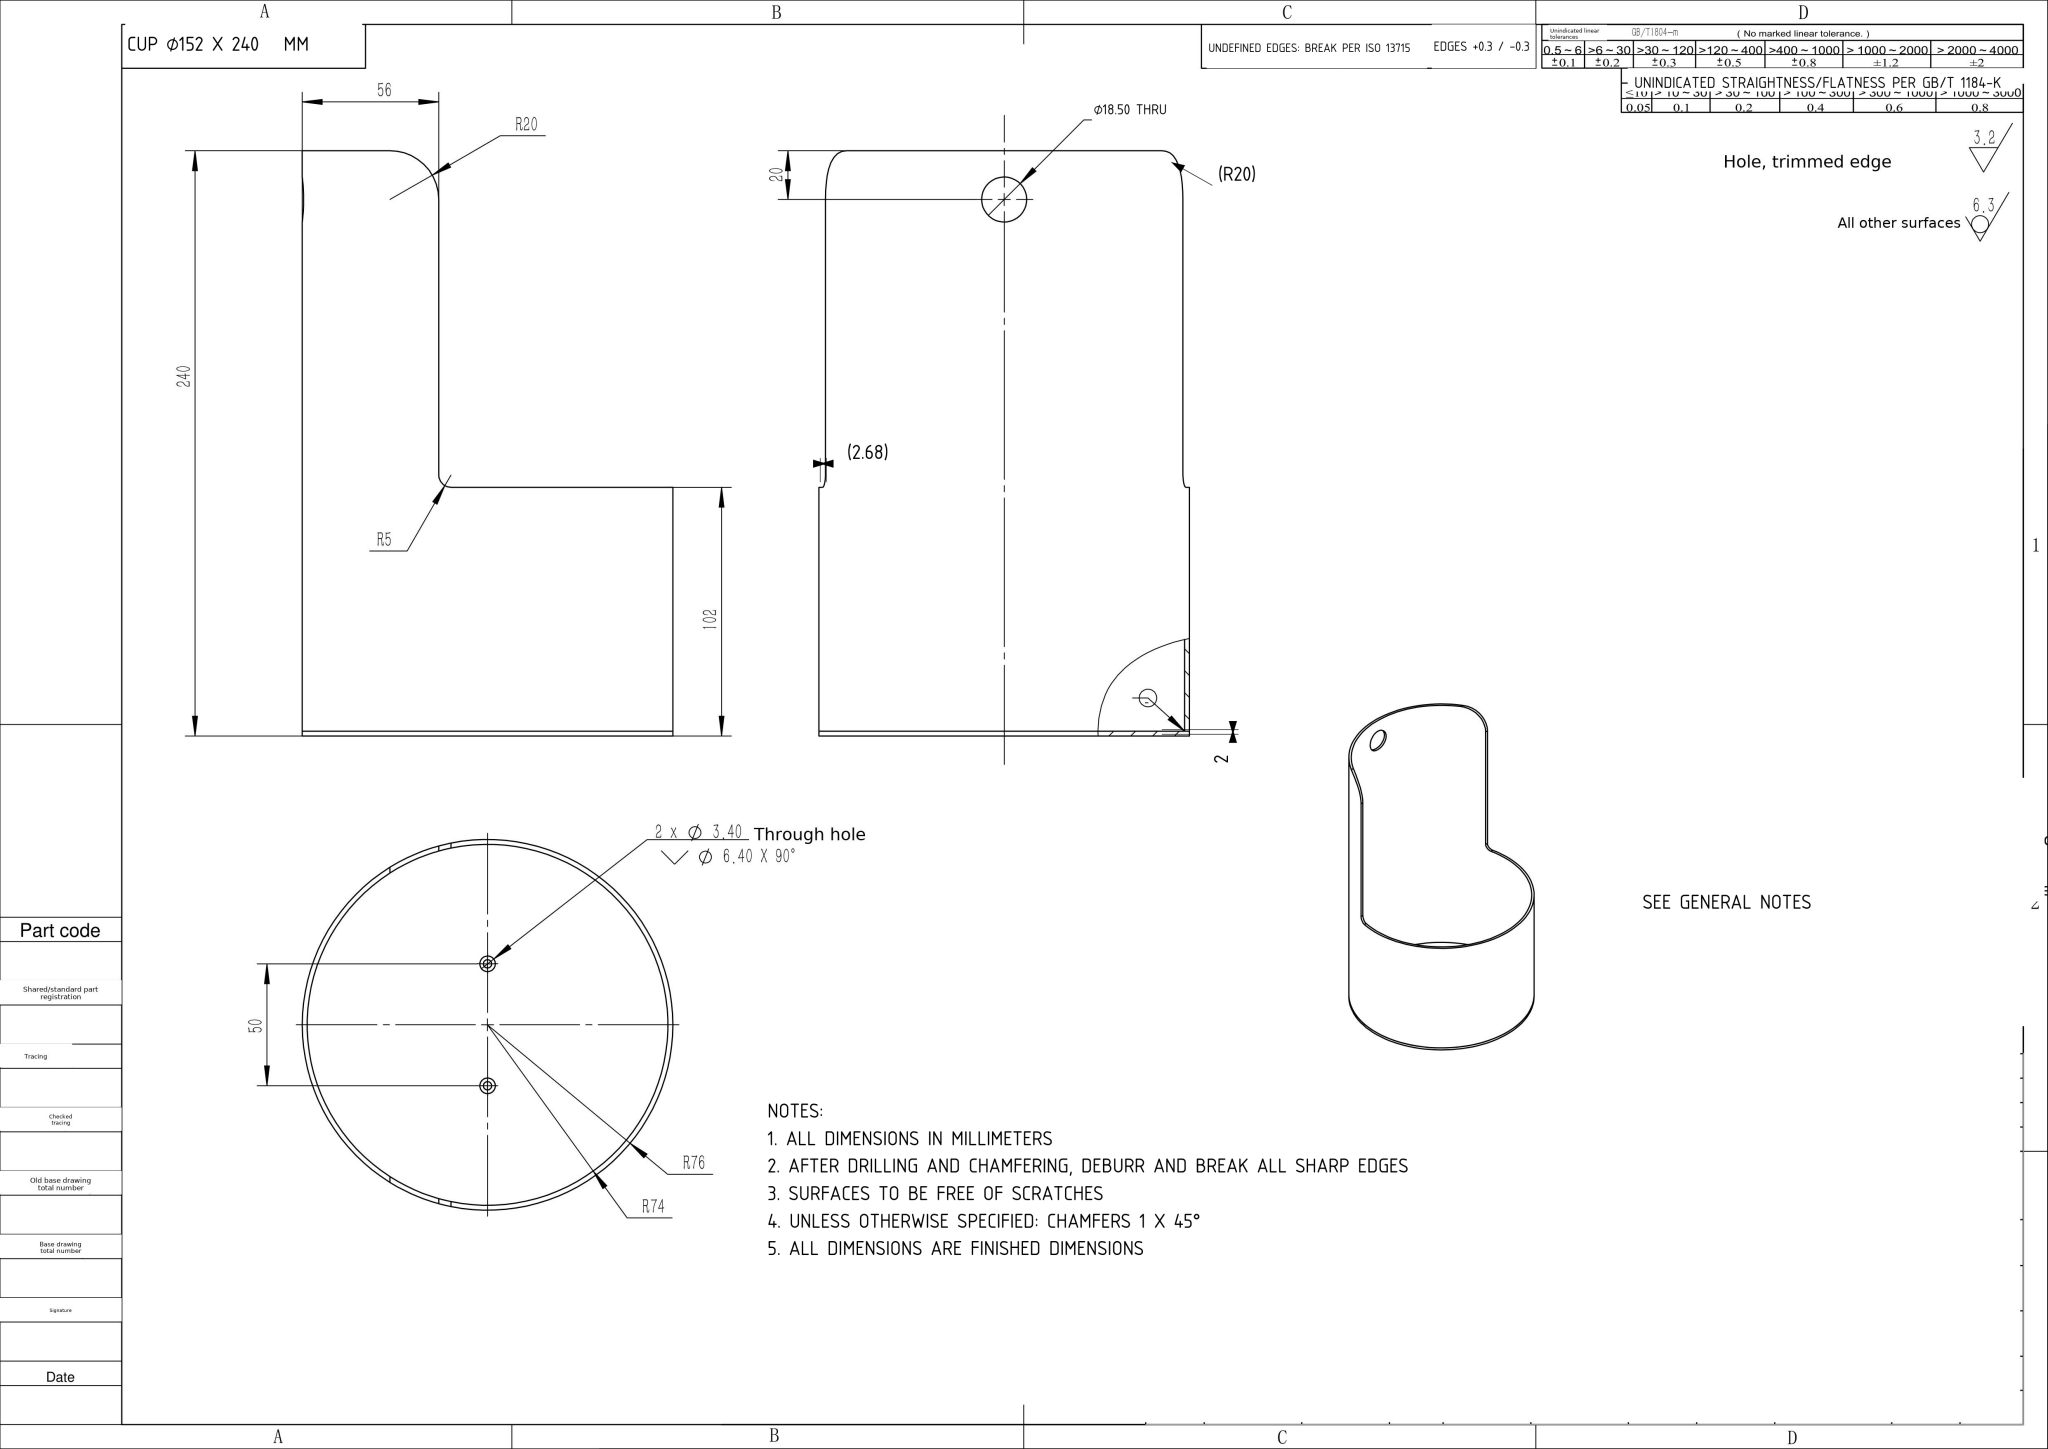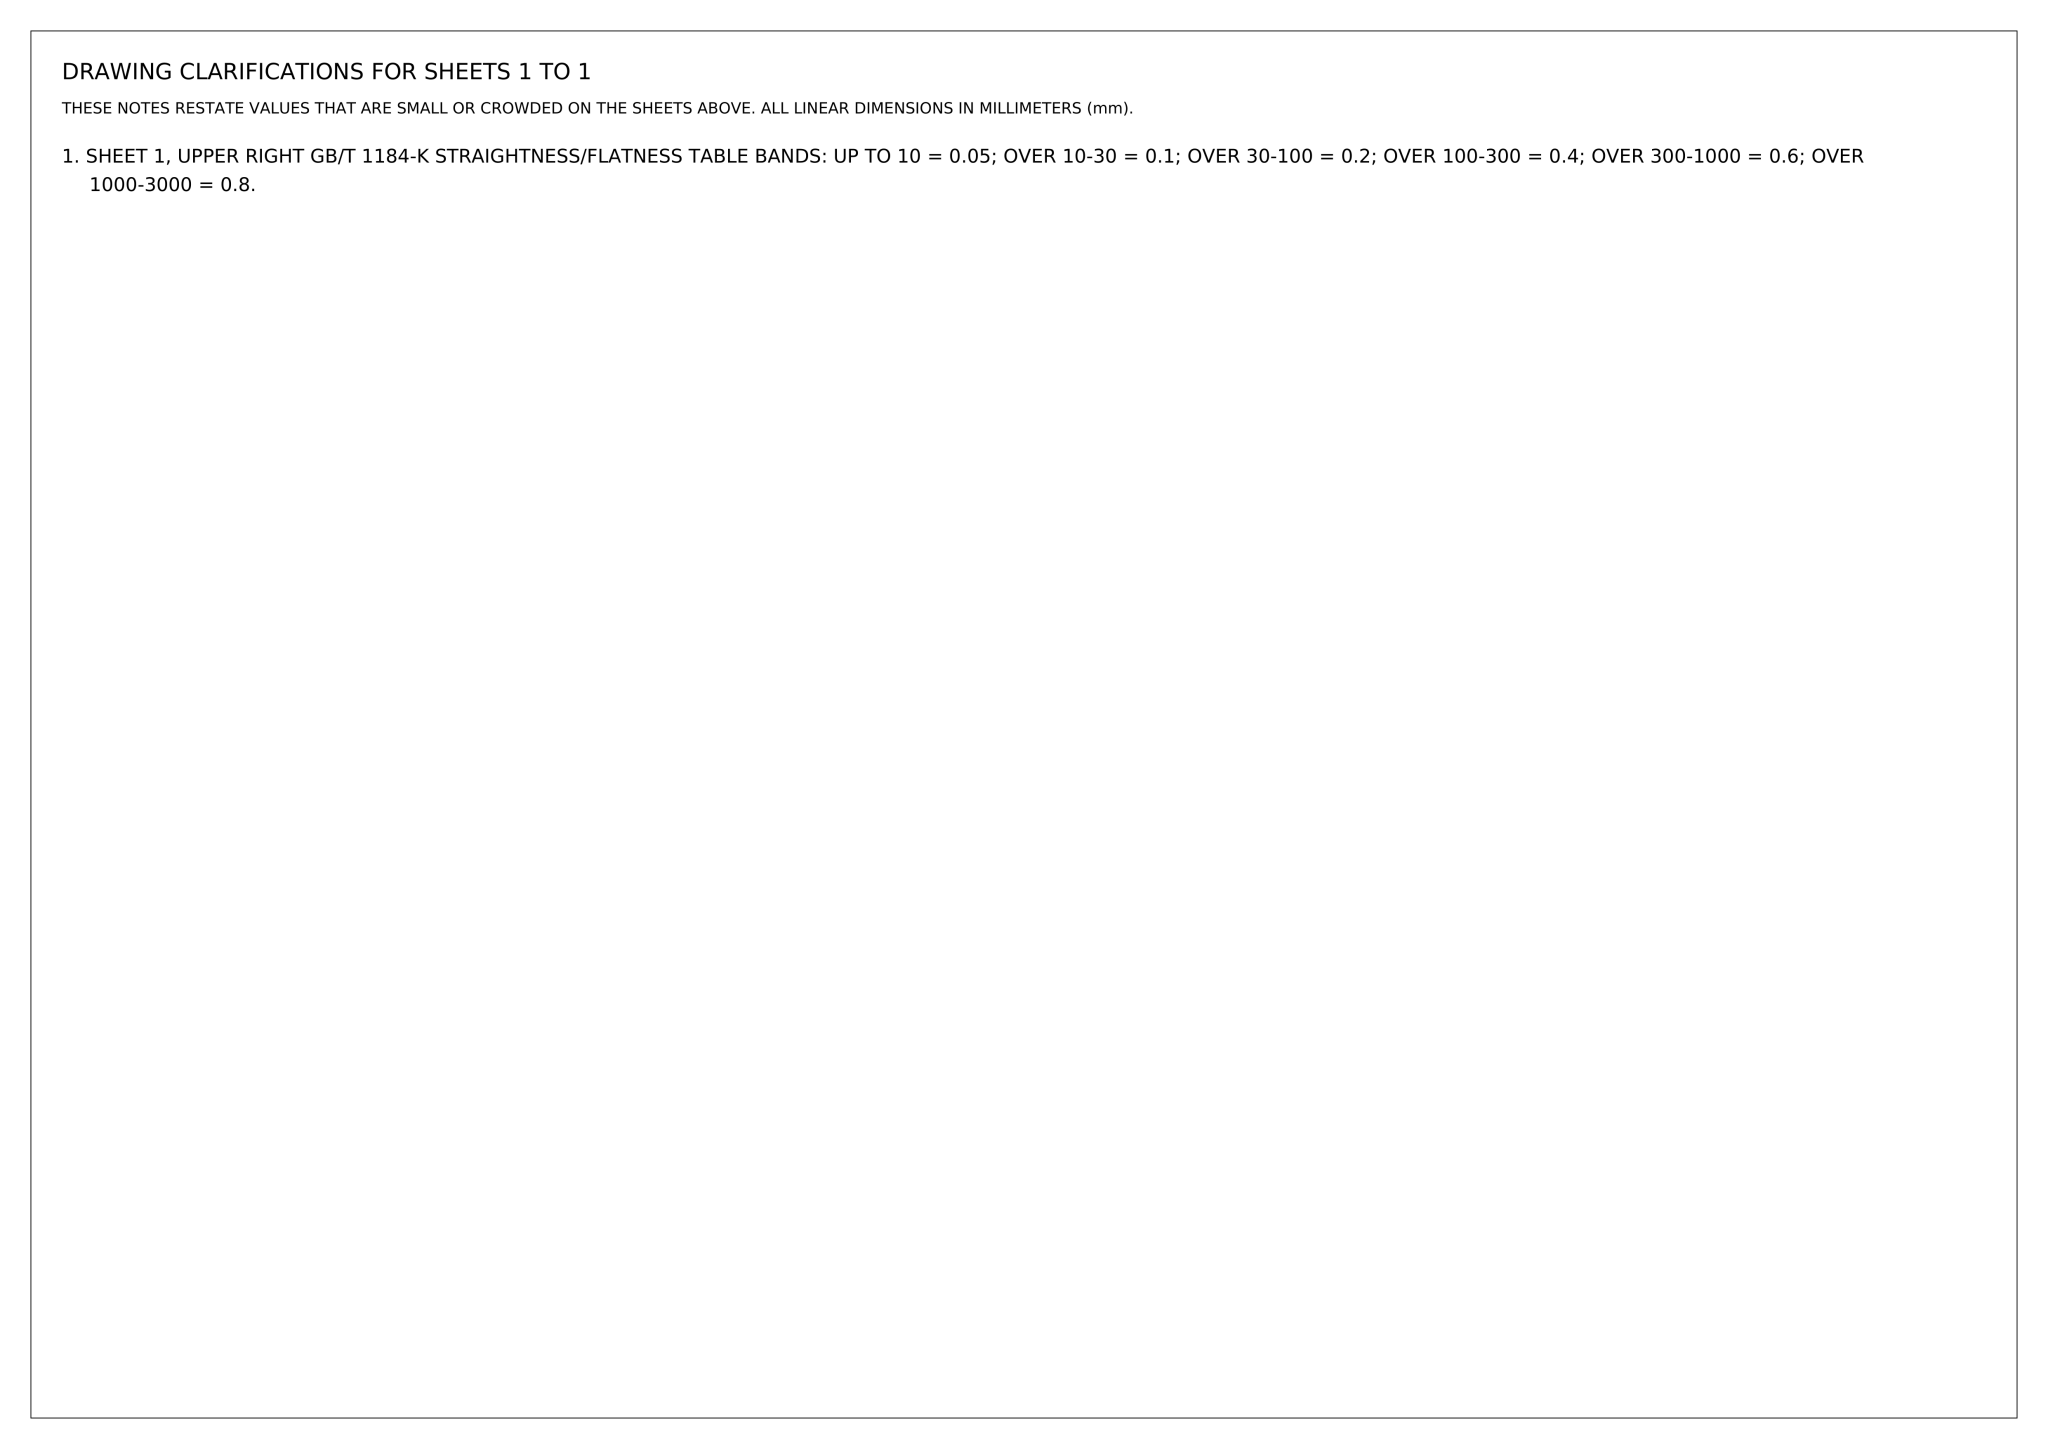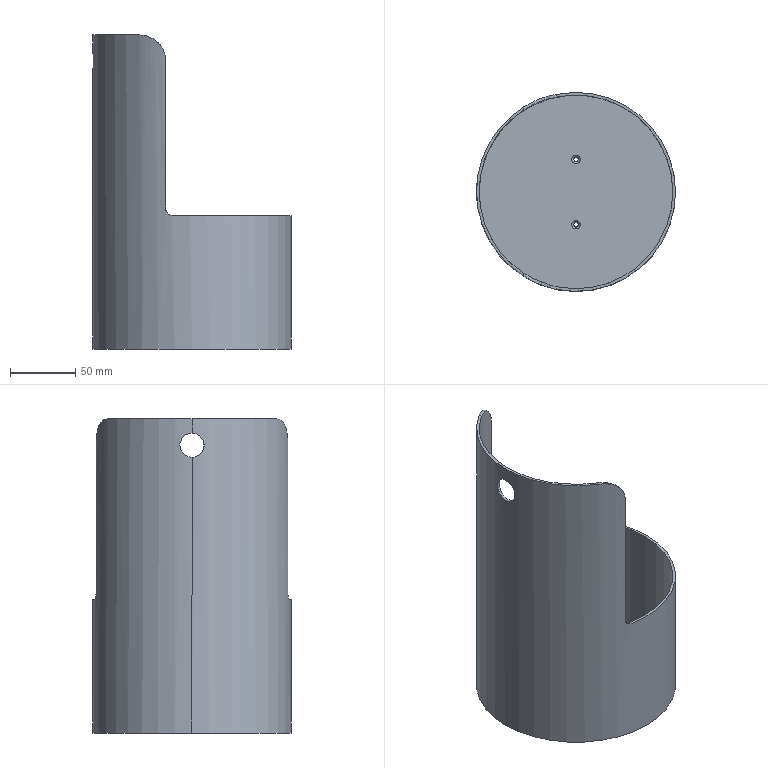Part | NX | mm | 1 solid | 24 faces | box 152 x 152 x 240 mm | volume 184378 mm3 | cylinder 14 | plane 6 | cone 4 | commonest cylinder face diameters 3.4 x4 18.5 x2 40 x2 10 x2 148 x2 152 x2